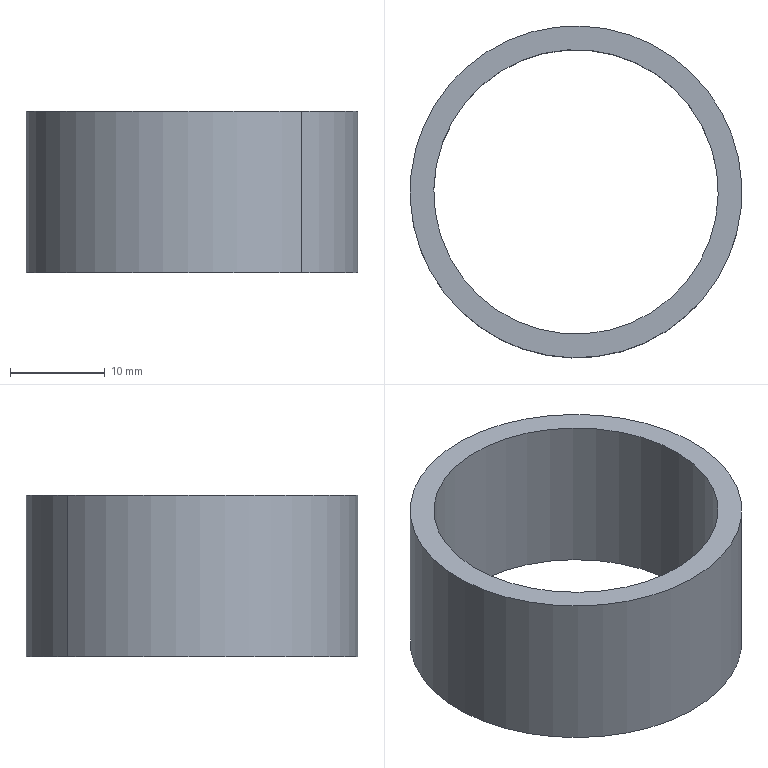Component | SolidWorks | -DrivePulleyStopSleeve-1 | 1 solid | 6 faces | box 35 x 35 x 17 mm | volume 4339 mm3 | cylinder 4 | plane 2 | commonest cylinder face diameters 30 x2 35 x2
build123d program:
from build123d import *

# Parameters (mm, degrees)
SKETCH1_R           = 17.5
SKETCH1_R_2         = 15
BOSS_EXTRUDE1_DEPTH = 8.5


with BuildPart() as part:
    # Sketch1 → Boss-Extrude1 (new, symmetric)
    with BuildSketch(Plane(origin=(0, 0, 0), x_dir=(0, 0, -1), z_dir=(1, 0, 0))):
        Circle(SKETCH1_R)
        Circle(SKETCH1_R_2, mode=Mode.SUBTRACT)
    extrude(amount=BOSS_EXTRUDE1_DEPTH, both=True)


solid = part.part

# Placed as in the assembly
solid = solid.moved(Location((205, 1094.5, 26.5), (0, 90, 0)))
STEP:
#1=COLOUR_RGB('',0.7922,0.8196,0.9333);
#2=FILL_AREA_STYLE_COLOUR('',#1);
#3=FILL_AREA_STYLE('',(#2));
#4=SURFACE_STYLE_FILL_AREA(#3);
#5=SURFACE_SIDE_STYLE('',(#4));
#6=SURFACE_STYLE_USAGE(.BOTH.,#5);
#7=PRESENTATION_STYLE_ASSIGNMENT((#6));
#8=CARTESIAN_POINT('',(7.68,43.533,0.7087));
#9=VERTEX_POINT('',#8);
#10=CARTESIAN_POINT('',(8.462,42.648,0.7087));
#11=VERTEX_POINT('',#10);
#12=CARTESIAN_POINT('',(8.071,43.091,0.7087));
#13=DIRECTION('',(-0.,-0.,-1.));
#14=DIRECTION('',(0.6622,-0.7493,-0.));
#15=AXIS2_PLACEMENT_3D('',#12,#13,#14);
#16=CIRCLE('',#15,0.5906);
#17=EDGE_CURVE('',#9,#11,#16,.T.);
#18=ORIENTED_EDGE('',*,*,#17,.T.);
#19=CARTESIAN_POINT('',(8.462,42.648,1.378));
#20=VERTEX_POINT('',#19);
#21=CARTESIAN_POINT('',(8.462,42.648,0.7087));
#22=DIRECTION('',(0.,0.,1.));
#23=VECTOR('',#22,39.37);
#24=LINE('',#21,#23);
#25=EDGE_CURVE('',#11,#20,#24,.T.);
#26=ORIENTED_EDGE('',*,*,#25,.T.);
#27=CARTESIAN_POINT('',(7.68,43.533,1.378));
#28=VERTEX_POINT('',#27);
#29=CARTESIAN_POINT('',(8.071,43.091,1.378));
#30=DIRECTION('',(-0.,-0.,-1.));
#31=DIRECTION('',(0.6622,-0.7493,0.));
#32=AXIS2_PLACEMENT_3D('',#29,#30,#31);
#33=CIRCLE('',#32,0.5906);
#34=EDGE_CURVE('',#28,#20,#33,.T.);
#35=ORIENTED_EDGE('',*,*,#34,.F.);
#36=CARTESIAN_POINT('',(7.68,43.533,0.7087));
#37=DIRECTION('',(0.,0.,1.));
#38=VECTOR('',#37,39.37);
#39=LINE('',#36,#38);
#40=EDGE_CURVE('',#9,#28,#39,.T.);
#41=ORIENTED_EDGE('',*,*,#40,.F.);
#42=EDGE_LOOP('',(#18,#26,#35,#41));
#43=FACE_OUTER_BOUND('',#42,.T.);
#44=CARTESIAN_POINT('',(8.071,43.091,0.7087));
#45=DIRECTION('',(0.,0.,1.));
#46=DIRECTION('',(-0.6622,0.7493,0.));
#47=AXIS2_PLACEMENT_3D('',#44,#45,#46);
#48=CYLINDRICAL_SURFACE('',#47,0.5906);
#49=ADVANCED_FACE('',(#43),#48,.F.);
#50=CARTESIAN_POINT('',(8.527,42.574,0.7087));
#51=VERTEX_POINT('',#50);
#52=CARTESIAN_POINT('',(7.615,43.607,0.7087));
#53=VERTEX_POINT('',#52);
#54=CARTESIAN_POINT('',(8.071,43.091,0.7087));
#55=DIRECTION('',(-0.,-0.,-1.));
#56=DIRECTION('',(0.6622,-0.7493,-0.));
#57=AXIS2_PLACEMENT_3D('',#54,#55,#56);
#58=CIRCLE('',#57,0.689);
#59=EDGE_CURVE('',#51,#53,#58,.T.);
#60=ORIENTED_EDGE('',*,*,#59,.F.);
#61=CARTESIAN_POINT('',(8.527,42.574,1.378));
#62=VERTEX_POINT('',#61);
#63=CARTESIAN_POINT('',(8.527,42.574,0.7087));
#64=DIRECTION('',(0.,0.,1.));
#65=VECTOR('',#64,39.37);
#66=LINE('',#63,#65);
#67=EDGE_CURVE('',#51,#62,#66,.T.);
#68=ORIENTED_EDGE('',*,*,#67,.T.);
#69=CARTESIAN_POINT('',(7.615,43.607,1.378));
#70=VERTEX_POINT('',#69);
#71=CARTESIAN_POINT('',(8.071,43.091,1.378));
#72=DIRECTION('',(-0.,-0.,-1.));
#73=DIRECTION('',(0.6622,-0.7493,0.));
#74=AXIS2_PLACEMENT_3D('',#71,#72,#73);
#75=CIRCLE('',#74,0.689);
#76=EDGE_CURVE('',#62,#70,#75,.T.);
#77=ORIENTED_EDGE('',*,*,#76,.T.);
#78=CARTESIAN_POINT('',(7.615,43.607,0.7087));
#79=DIRECTION('',(0.,0.,1.));
#80=VECTOR('',#79,39.37);
#81=LINE('',#78,#80);
#82=EDGE_CURVE('',#53,#70,#81,.T.);
#83=ORIENTED_EDGE('',*,*,#82,.F.);
#84=EDGE_LOOP('',(#60,#68,#77,#83));
#85=FACE_OUTER_BOUND('',#84,.T.);
#86=CARTESIAN_POINT('',(8.071,43.091,0.7087));
#87=DIRECTION('',(0.,0.,1.));
#88=DIRECTION('',(-0.6622,0.7493,0.));
#89=AXIS2_PLACEMENT_3D('',#86,#87,#88);
#90=CYLINDRICAL_SURFACE('',#89,0.689);
#91=ADVANCED_FACE('',(#85),#90,.T.);
#92=CARTESIAN_POINT('',(8.071,43.091,0.7087));
#93=DIRECTION('',(-0.,-0.,-1.));
#94=DIRECTION('',(0.6622,-0.7493,-0.));
#95=AXIS2_PLACEMENT_3D('',#92,#93,#94);
#96=CIRCLE('',#95,0.689);
#97=EDGE_CURVE('',#53,#51,#96,.T.);
#98=ORIENTED_EDGE('',*,*,#97,.T.);
#99=ORIENTED_EDGE('',*,*,#59,.T.);
#100=EDGE_LOOP('',(#98,#99));
#101=FACE_OUTER_BOUND('',#100,.T.);
#102=ORIENTED_EDGE('',*,*,#17,.F.);
#103=CARTESIAN_POINT('',(8.071,43.091,0.7087));
#104=DIRECTION('',(-0.,-0.,-1.));
#105=DIRECTION('',(0.6622,-0.7493,-0.));
#106=AXIS2_PLACEMENT_3D('',#103,#104,#105);
#107=CIRCLE('',#106,0.5906);
#108=EDGE_CURVE('',#11,#9,#107,.T.);
#109=ORIENTED_EDGE('',*,*,#108,.F.);
#110=EDGE_LOOP('',(#102,#109));
#111=FACE_BOUND('',#110,.T.);
#112=CARTESIAN_POINT('',(8.071,43.091,0.7087));
#113=DIRECTION('',(-0.,-0.,-1.));
#114=DIRECTION('',(0.6622,-0.7493,-0.));
#115=AXIS2_PLACEMENT_3D('',#112,#113,#114);
#116=PLANE('',#115);
#117=ADVANCED_FACE('',(#101,#111),#116,.T.);
#118=CARTESIAN_POINT('',(8.071,43.091,1.378));
#119=DIRECTION('',(-0.,-0.,-1.));
#120=DIRECTION('',(0.6622,-0.7493,0.));
#121=AXIS2_PLACEMENT_3D('',#118,#119,#120);
#122=CIRCLE('',#121,0.689);
#123=EDGE_CURVE('',#70,#62,#122,.T.);
#124=ORIENTED_EDGE('',*,*,#123,.F.);
#125=ORIENTED_EDGE('',*,*,#76,.F.);
#126=EDGE_LOOP('',(#124,#125));
#127=FACE_OUTER_BOUND('',#126,.T.);
#128=ORIENTED_EDGE('',*,*,#34,.T.);
#129=CARTESIAN_POINT('',(8.071,43.091,1.378));
#130=DIRECTION('',(-0.,-0.,-1.));
#131=DIRECTION('',(0.6622,-0.7493,0.));
#132=AXIS2_PLACEMENT_3D('',#129,#130,#131);
#133=CIRCLE('',#132,0.5906);
#134=EDGE_CURVE('',#20,#28,#133,.T.);
#135=ORIENTED_EDGE('',*,*,#134,.T.);
#136=EDGE_LOOP('',(#128,#135));
#137=FACE_BOUND('',#136,.T.);
#138=CARTESIAN_POINT('',(8.071,43.091,1.378));
#139=DIRECTION('',(-0.,-0.,-1.));
#140=DIRECTION('',(0.6622,-0.7493,-0.));
#141=AXIS2_PLACEMENT_3D('',#138,#139,#140);
#142=PLANE('',#141);
#143=ADVANCED_FACE('',(#127,#137),#142,.F.);
#144=ORIENTED_EDGE('',*,*,#67,.F.);
#145=ORIENTED_EDGE('',*,*,#97,.F.);
#146=ORIENTED_EDGE('',*,*,#82,.T.);
#147=ORIENTED_EDGE('',*,*,#123,.T.);
#148=EDGE_LOOP('',(#144,#145,#146,#147));
#149=FACE_OUTER_BOUND('',#148,.T.);
#150=CARTESIAN_POINT('',(8.071,43.091,0.7087));
#151=DIRECTION('',(0.,0.,1.));
#152=DIRECTION('',(-0.6622,0.7493,0.));
#153=AXIS2_PLACEMENT_3D('',#150,#151,#152);
#154=CYLINDRICAL_SURFACE('',#153,0.689);
#155=ADVANCED_FACE('',(#149),#154,.T.);
#156=ORIENTED_EDGE('',*,*,#25,.F.);
#157=ORIENTED_EDGE('',*,*,#108,.T.);
#158=ORIENTED_EDGE('',*,*,#40,.T.);
#159=ORIENTED_EDGE('',*,*,#134,.F.);
#160=EDGE_LOOP('',(#156,#157,#158,#159));
#161=FACE_OUTER_BOUND('',#160,.T.);
#162=CARTESIAN_POINT('',(8.071,43.091,0.7087));
#163=DIRECTION('',(0.,0.,1.));
#164=DIRECTION('',(-0.6622,0.7493,0.));
#165=AXIS2_PLACEMENT_3D('',#162,#163,#164);
#166=CYLINDRICAL_SURFACE('',#165,0.5906);
#167=ADVANCED_FACE('',(#161),#166,.F.);
#168=CLOSED_SHELL('',(#49,#91,#117,#143,#155,#167));
#169=MANIFOLD_SOLID_BREP('',#168);
#170=STYLED_ITEM('',(#7),#169);
#171=PRESENTATION_LAYER_ASSIGNMENT('','',(#170));
#172=CARTESIAN_POINT('',(0.,0.,0.));
#173=DIRECTION('',(0.,0.,1.));
#174=DIRECTION('',(1.,0.,0.));
#175=AXIS2_PLACEMENT_3D('',#172,#173,#174);
#176=(LENGTH_UNIT()NAMED_UNIT(*)SI_UNIT($,.METRE.));
#177=LENGTH_MEASURE_WITH_UNIT(LENGTH_MEASURE(0.0254),#176);
#178=DIMENSIONAL_EXPONENTS(1.,0.,0.,0.,0.,0.,0.);
#179=(CONVERSION_BASED_UNIT('',#177)LENGTH_UNIT()NAMED_UNIT(#178));
#180=UNCERTAINTY_MEASURE_WITH_UNIT(LENGTH_MEASURE(0.00001),#179,'','');
#181=(NAMED_UNIT(*)PLANE_ANGLE_UNIT()SI_UNIT($,.RADIAN.));
#182=(NAMED_UNIT(*)SI_UNIT($,.STERADIAN.)SOLID_ANGLE_UNIT());
#183=(GEOMETRIC_REPRESENTATION_CONTEXT(3)GLOBAL_UNCERTAINTY_ASSIGNED_CONTEXT((#180))GLOBAL_UNIT_ASSIGNED_CONTEXT((#179,#181,#182))REPRESENTATION_CONTEXT('',''));
#184=ADVANCED_BREP_SHAPE_REPRESENTATION('',(#169,#175),#183);
#185=(LENGTH_UNIT()NAMED_UNIT(*)SI_UNIT($,.METRE.));
#186=LENGTH_MEASURE_WITH_UNIT(LENGTH_MEASURE(0.0254),#185);
#187=DIMENSIONAL_EXPONENTS(1.,0.,0.,0.,0.,0.,0.);
#188=(CONVERSION_BASED_UNIT('',#186)LENGTH_UNIT()NAMED_UNIT(#187));
#189=UNCERTAINTY_MEASURE_WITH_UNIT(LENGTH_MEASURE(0.00001),#188,'','');
#190=(NAMED_UNIT(*)PLANE_ANGLE_UNIT()SI_UNIT($,.RADIAN.));
#191=(NAMED_UNIT(*)SI_UNIT($,.STERADIAN.)SOLID_ANGLE_UNIT());
#192=(GEOMETRIC_REPRESENTATION_CONTEXT(3)GLOBAL_UNCERTAINTY_ASSIGNED_CONTEXT((#189))GLOBAL_UNIT_ASSIGNED_CONTEXT((#188,#190,#191))REPRESENTATION_CONTEXT('',''));
#193=MECHANICAL_DESIGN_GEOMETRIC_PRESENTATION_REPRESENTATION('',(#170),#192);